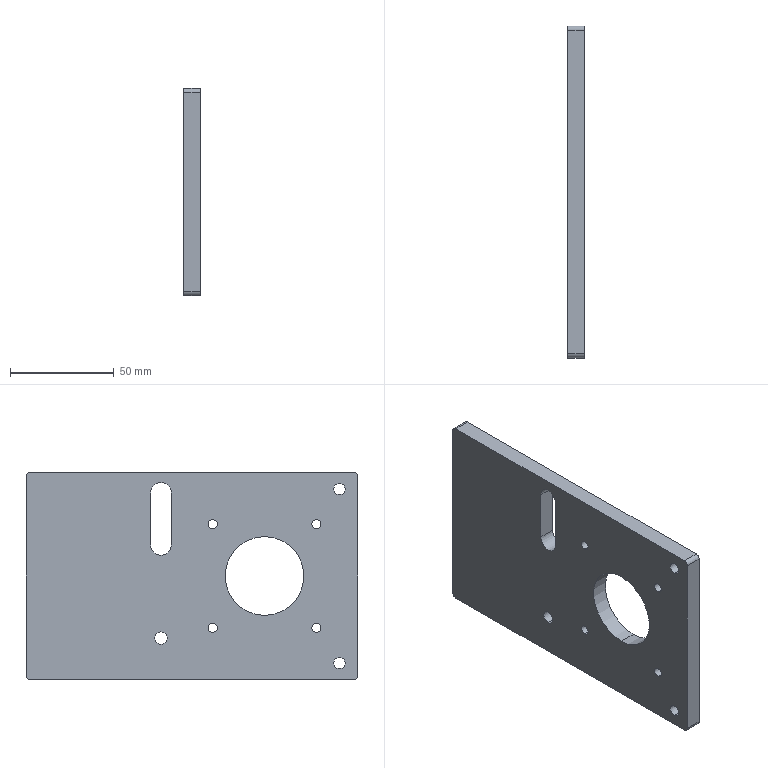Component | SolidWorks | CHEN123-AA-12-1 | 1 solid | 43 faces | box 8 x 160 x 100 mm | volume 114551 mm3 | cylinder 31 | plane 12 | commonest cylinder face diameters 8 x8 4.5 x8 5.5 x4 4 x4 10 x3 6 x2 38 x2
build123d program:
from build123d import *

# Parameters (mm, degrees)
SKETCH1_W                                       = 100
SKETCH1_H                                       = 160
BOSS_EXTRUDE1_DEPTH                             = 8
FILLET1_R                                       = 2
SKETCH2_R                                       = 19
CUT_EXTRUDE1_DEPTH                              = 20
SKETCH3_R                                       = 3
CUT_EXTRUDE2_DEPTH                              = 95.678
F_5_5_5_5_DIAMETER_HOLE1_D                      = 5.5
F_5_5_5_5_DIAMETER_HOLE1_DEPTH                  = 10.1
F_5_5_5_5_DIAMETER_HOLE1_TIP                    = 1.652
M4_HEX_SOCKET_HEAD_CAP_SCREW_CBORE1_D           = 4.5
M4_HEX_SOCKET_HEAD_CAP_SCREW_CBORE1_CBORE_D     = 8
M4_HEX_SOCKET_HEAD_CAP_SCREW_CBORE1_CBORE_DEPTH = 4.4


with BuildPart() as part:
    # Sketch1 → Boss-Extrude1 (new body)
    with BuildSketch(Plane.XY):
        Rectangle(SKETCH1_W, SKETCH1_H)
    extrude(amount=BOSS_EXTRUDE1_DEPTH)

    # Fillet1
    fillet1_edges = [part.edges().sort_by_distance(p)[0] for p in [
        (50, -80, 4),
        (-50, -80, 4),
        (-50, 80, 4),
        (50, 80, 4),
    ]]
    fillet(fillet1_edges, radius=FILLET1_R)

    # Sketch2 → Cut-Extrude1 (cut)
    with BuildSketch(Plane(origin=(0, 0, 0), x_dir=(-1, 0, 0), z_dir=(0, 0, -1))):
        with Locations((0, -35)):
            Circle(SKETCH2_R)
    extrude(amount=-CUT_EXTRUDE1_DEPTH, mode=Mode.SUBTRACT)

    # Sketch3 → Cut-Extrude2 (cut, through all)
    with BuildSketch(Plane(origin=(0, 0, 0), x_dir=(-1, 0, 0), z_dir=(0, 0, -1))):
        with Locations((-30, 15)):
            Circle(SKETCH3_R)
        with BuildLine():
            Line((40, 10), (15, 10))
            ThreePointArc((15, 10), (10, 15), (15, 20))
            Line((15, 20), (40, 20))
            ThreePointArc((40, 20), (45, 15), (40, 10))
        make_face()
    extrude(amount=-CUT_EXTRUDE2_DEPTH, mode=Mode.SUBTRACT)

    # 5.5 _5.5_ Diameter Hole1
    with Locations(Plane(origin=(0, 0, 0), x_dir=(-1, 0, 0), z_dir=(0, 0, -1))):
        with Locations((-42.036, -71.098), (41.933, -71.098)):
            Hole(F_5_5_5_5_DIAMETER_HOLE1_D / 2, depth=F_5_5_5_5_DIAMETER_HOLE1_DEPTH)
            with Locations((0, 0, -(F_5_5_5_5_DIAMETER_HOLE1_DEPTH + F_5_5_5_5_DIAMETER_HOLE1_TIP / 2))):  # 118° drill point
                Cone(0, F_5_5_5_5_DIAMETER_HOLE1_D / 2, F_5_5_5_5_DIAMETER_HOLE1_TIP, mode=Mode.SUBTRACT)

    # M4 Hex Socket Head Cap Screw CBORE1 (through all)
    with Locations(Plane.XY.offset(8)):
        with Locations((-25, -60), (-25, -10), (25, -60), (25, -10)):
            CounterBoreHole(M4_HEX_SOCKET_HEAD_CAP_SCREW_CBORE1_D / 2, M4_HEX_SOCKET_HEAD_CAP_SCREW_CBORE1_CBORE_D / 2, M4_HEX_SOCKET_HEAD_CAP_SCREW_CBORE1_CBORE_DEPTH)


solid = part.part

# Placed as in the assembly
solid = solid.moved(Location((-28, -60.999, -200), (0, 90, 0)))